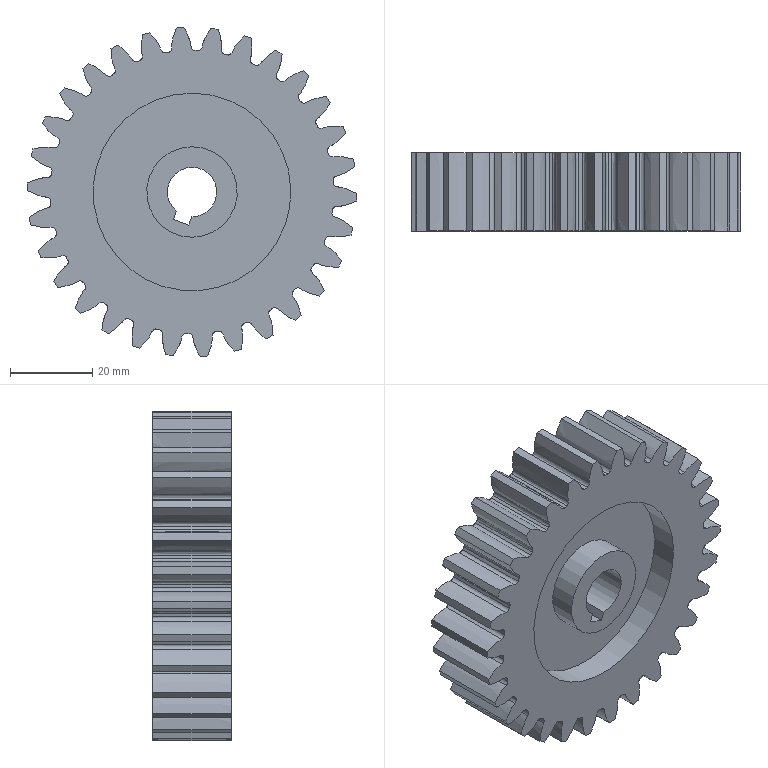Component | NX | 4 | 1 solid | 194 faces | volume 62171 mm3 | other 150 | cylinder 35 | plane 9 | commonest cylinder face diameters 68.75 x30 48 x2 22 x2 12 x1